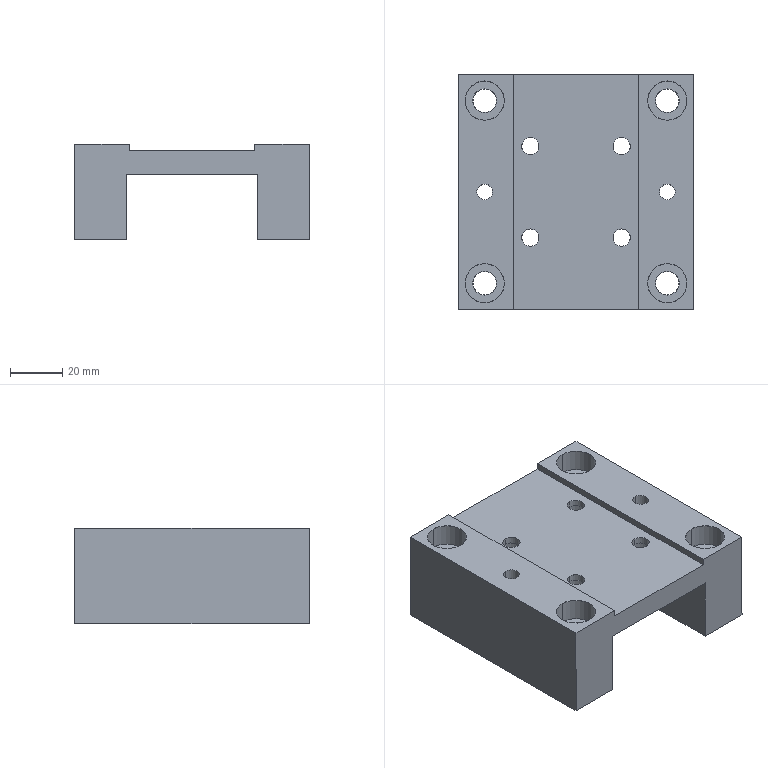Component | SolidWorks | Y-AxisSliderRiserBlock-1 | 1 solid | 106 faces | box 90 x 90 x 36.5 mm | volume 154318 mm3 | cone 48 | cylinder 36 | plane 22 | commonest cylinder face diameters 15 x8 9 x8 11 x8 6.6 x8 6 x4
build123d program:
from build123d import *

# Parameters (mm, degrees)
SKETCH1_W                                      = 90
SKETCH1_H                                      = 90
BOSS_EXTRUDE1_DEPTH                            = 36.5
SKETCH2_W                                      = 90
SKETCH2_H                                      = 48
CUT_EXTRUDE1_DEPTH                             = 2.5
SKETCH9_W                                      = 50
SKETCH9_H                                      = 50
CUT_EXTRUDE2_DEPTH                             = 108.039
M6_HEX_SOCKET_HEAD_CAP_SCREW_CBORE1_AT_2_COUNT = 2
M6_HEX_SOCKET_HEAD_CAP_SCREW_CBORE1_AT_2_PITCH = 35
M6_HEX_SOCKET_HEAD_CAP_SCREW_CBORE1_AT_3_COUNT = 2
M6_HEX_SOCKET_HEAD_CAP_SCREW_CBORE1_AT_3_PITCH = 49.497
M6_HEX_SOCKET_HEAD_CAP_SCREW_CBORE1_AT_4_COUNT = 2
M6_HEX_SOCKET_HEAD_CAP_SCREW_CBORE1_AT_4_PITCH = 35
M8_HEX_SOCKET_HEAD_CAP_SCREW_CBORE1_AT_2_COUNT = 2
M8_HEX_SOCKET_HEAD_CAP_SCREW_CBORE1_AT_2_PITCH = 70
M8_HEX_SOCKET_HEAD_CAP_SCREW_CBORE1_AT_3_COUNT = 2
M8_HEX_SOCKET_HEAD_CAP_SCREW_CBORE1_AT_3_PITCH = 98.995
M8_HEX_SOCKET_HEAD_CAP_SCREW_CBORE1_AT_4_COUNT = 2
M8_HEX_SOCKET_HEAD_CAP_SCREW_CBORE1_AT_4_PITCH = 70
SKETCH6_R                                      = 3
CUT_EXTRUDE3_DEPTH                             = 74.364


with BuildPart() as part:
    # Sketch1 → Boss-Extrude1 (new body)
    with BuildSketch(Plane.XY):
        Rectangle(SKETCH1_W, SKETCH1_H)
    extrude(amount=BOSS_EXTRUDE1_DEPTH)

    # Sketch2 → Cut-Extrude1 (cut)
    with BuildSketch(Plane.XY.offset(36.5)):
        Rectangle(SKETCH2_W, SKETCH2_H)
    extrude(amount=-CUT_EXTRUDE1_DEPTH, mode=Mode.SUBTRACT)

    # Sketch9 → Cut-Extrude2 (cut, through all)
    with BuildSketch(Plane(origin=(45, 0, 0), x_dir=(0, 0, -1), z_dir=(1, 0, 0))):
        Rectangle(SKETCH9_W, SKETCH9_H)
    extrude(amount=-CUT_EXTRUDE2_DEPTH, mode=Mode.SUBTRACT)

    # Sketch4 → M6 Hex Socket Head Cap Screw CBORE1 (revolve, cut)
    with BuildSketch(Plane(origin=(17.5, 17.5, 25), x_dir=(0, 1, 0), z_dir=(1, 0, 0))):
        Polygon((0, 0), (0, 9), (3.325, 9), (3.3, 8.975), (3.3, 6.425), (3.325, 6.4), (5.5, 6.4), (5.5, 0.025), (5.525, 0), align=None)
    m6_hex_socket_head_cap_screw_cbore1 = revolve(axis=Axis((17.5, 17.5, 18.65), (0, 0, 1)), mode=Mode.SUBTRACT)

    # M6 Hex Socket Head Cap Screw CBORE1 at 2: M6 Hex Socket Head Cap Screw CBORE1 ×2
    with Locations(*[(-i * M6_HEX_SOCKET_HEAD_CAP_SCREW_CBORE1_AT_2_PITCH, 0, 0) for i in range(1, M6_HEX_SOCKET_HEAD_CAP_SCREW_CBORE1_AT_2_COUNT)]):
        add(m6_hex_socket_head_cap_screw_cbore1, mode=Mode.SUBTRACT)

    # M6 Hex Socket Head Cap Screw CBORE1 at 3: M6 Hex Socket Head Cap Screw CBORE1 ×2
    with Locations(*[Vector(-0.7071, -0.7071, 0) * (i * M6_HEX_SOCKET_HEAD_CAP_SCREW_CBORE1_AT_3_PITCH) for i in range(1, M6_HEX_SOCKET_HEAD_CAP_SCREW_CBORE1_AT_3_COUNT)]):
        add(m6_hex_socket_head_cap_screw_cbore1, mode=Mode.SUBTRACT)

    # M6 Hex Socket Head Cap Screw CBORE1 at 4: M6 Hex Socket Head Cap Screw CBORE1 ×2
    with Locations(*[(0, -i * M6_HEX_SOCKET_HEAD_CAP_SCREW_CBORE1_AT_4_PITCH, 0) for i in range(1, M6_HEX_SOCKET_HEAD_CAP_SCREW_CBORE1_AT_4_COUNT)]):
        add(m6_hex_socket_head_cap_screw_cbore1, mode=Mode.SUBTRACT)

    # Sketch7 → M8 Hex Socket Head Cap Screw CBORE1 (revolve, cut)
    with BuildSketch(Plane(origin=(-35, 35, 36.5), x_dir=(0, -1, 0), z_dir=(1, 0, 0))):
        Polygon((0, 0), (0, 36.5), (4.525, 36.5), (4.5, 36.475), (4.5, 8.625), (4.525, 8.6), (7.5, 8.6), (7.5, 0.025), (7.525, 0), align=None)
    m8_hex_socket_head_cap_screw_cbore1 = revolve(axis=Axis((-35, 35, 42.85), (0, 0, -1)), mode=Mode.SUBTRACT)

    # M8 Hex Socket Head Cap Screw CBORE1 at 2: M8 Hex Socket Head Cap Screw CBORE1 ×2
    with Locations(*[(i * M8_HEX_SOCKET_HEAD_CAP_SCREW_CBORE1_AT_2_PITCH, 0, 0) for i in range(1, M8_HEX_SOCKET_HEAD_CAP_SCREW_CBORE1_AT_2_COUNT)]):
        add(m8_hex_socket_head_cap_screw_cbore1, mode=Mode.SUBTRACT)

    # M8 Hex Socket Head Cap Screw CBORE1 at 3: M8 Hex Socket Head Cap Screw CBORE1 ×2
    with Locations(*[Vector(0.7071, -0.7071, 0) * (i * M8_HEX_SOCKET_HEAD_CAP_SCREW_CBORE1_AT_3_PITCH) for i in range(1, M8_HEX_SOCKET_HEAD_CAP_SCREW_CBORE1_AT_3_COUNT)]):
        add(m8_hex_socket_head_cap_screw_cbore1, mode=Mode.SUBTRACT)

    # M8 Hex Socket Head Cap Screw CBORE1 at 4: M8 Hex Socket Head Cap Screw CBORE1 ×2
    with Locations(*[(0, -i * M8_HEX_SOCKET_HEAD_CAP_SCREW_CBORE1_AT_4_PITCH, 0) for i in range(1, M8_HEX_SOCKET_HEAD_CAP_SCREW_CBORE1_AT_4_COUNT)]):
        add(m8_hex_socket_head_cap_screw_cbore1, mode=Mode.SUBTRACT)

    # Sketch6 → Cut-Extrude3 (cut, through all)
    with BuildSketch(Plane.XY.offset(36.5)):
        with Locations((0, 35)):
            Circle(SKETCH6_R)
        with Locations((0, -35)):
            Circle(SKETCH6_R)
    extrude(amount=-CUT_EXTRUDE3_DEPTH, mode=Mode.SUBTRACT)


solid = part.part

# Placed as in the assembly
solid = solid.moved(Location((90.729, -71.882, -98.5), (0, 0, 90)))